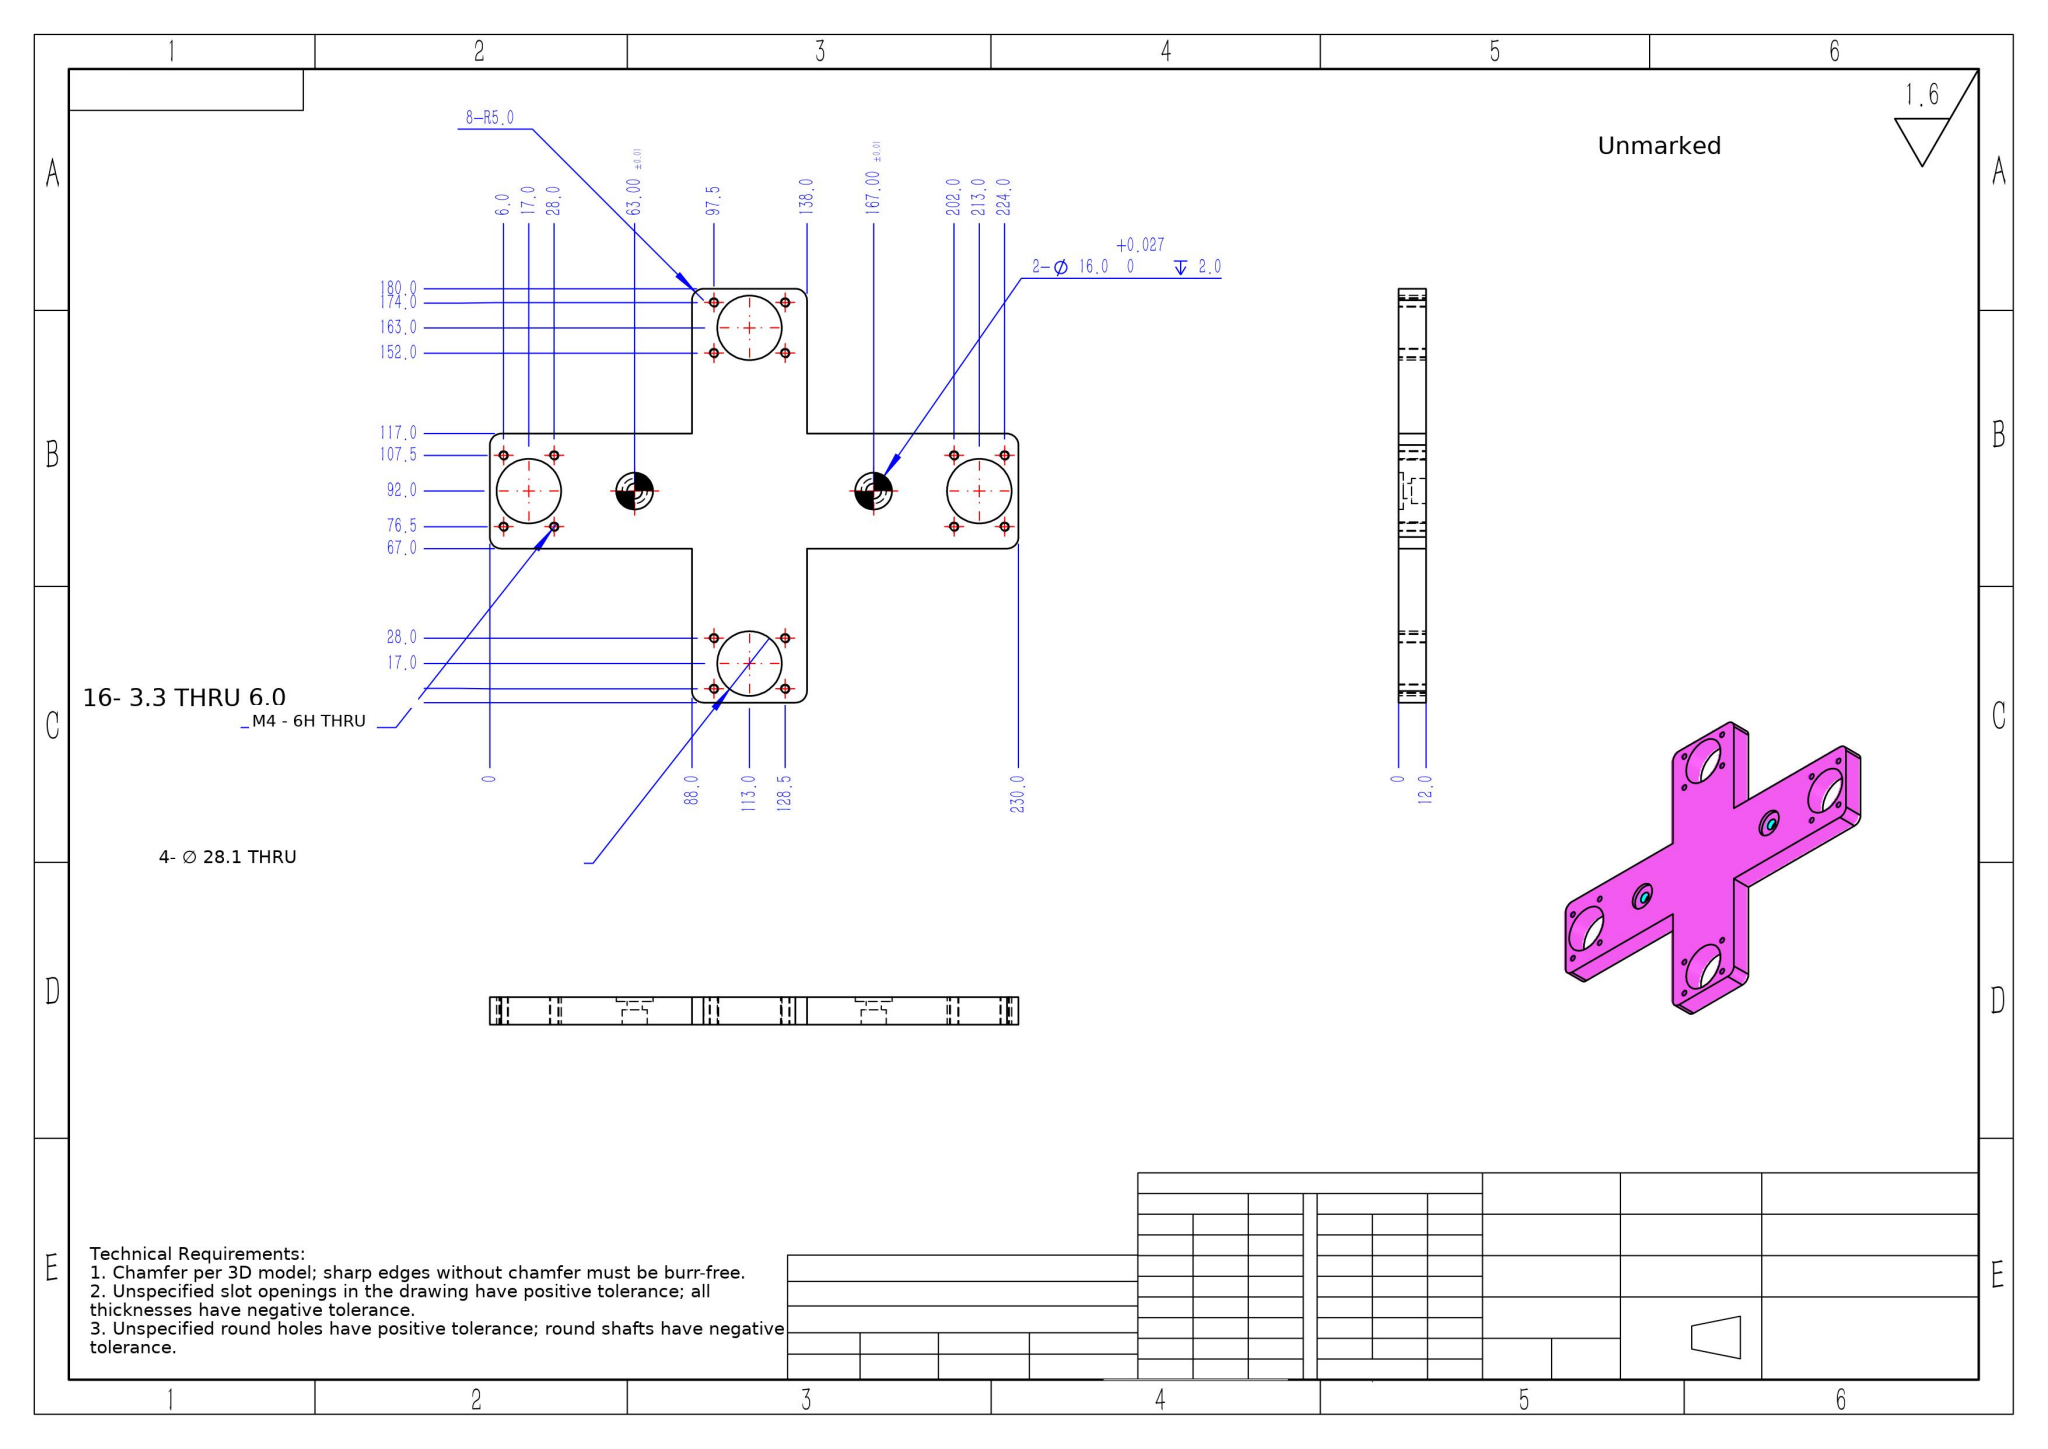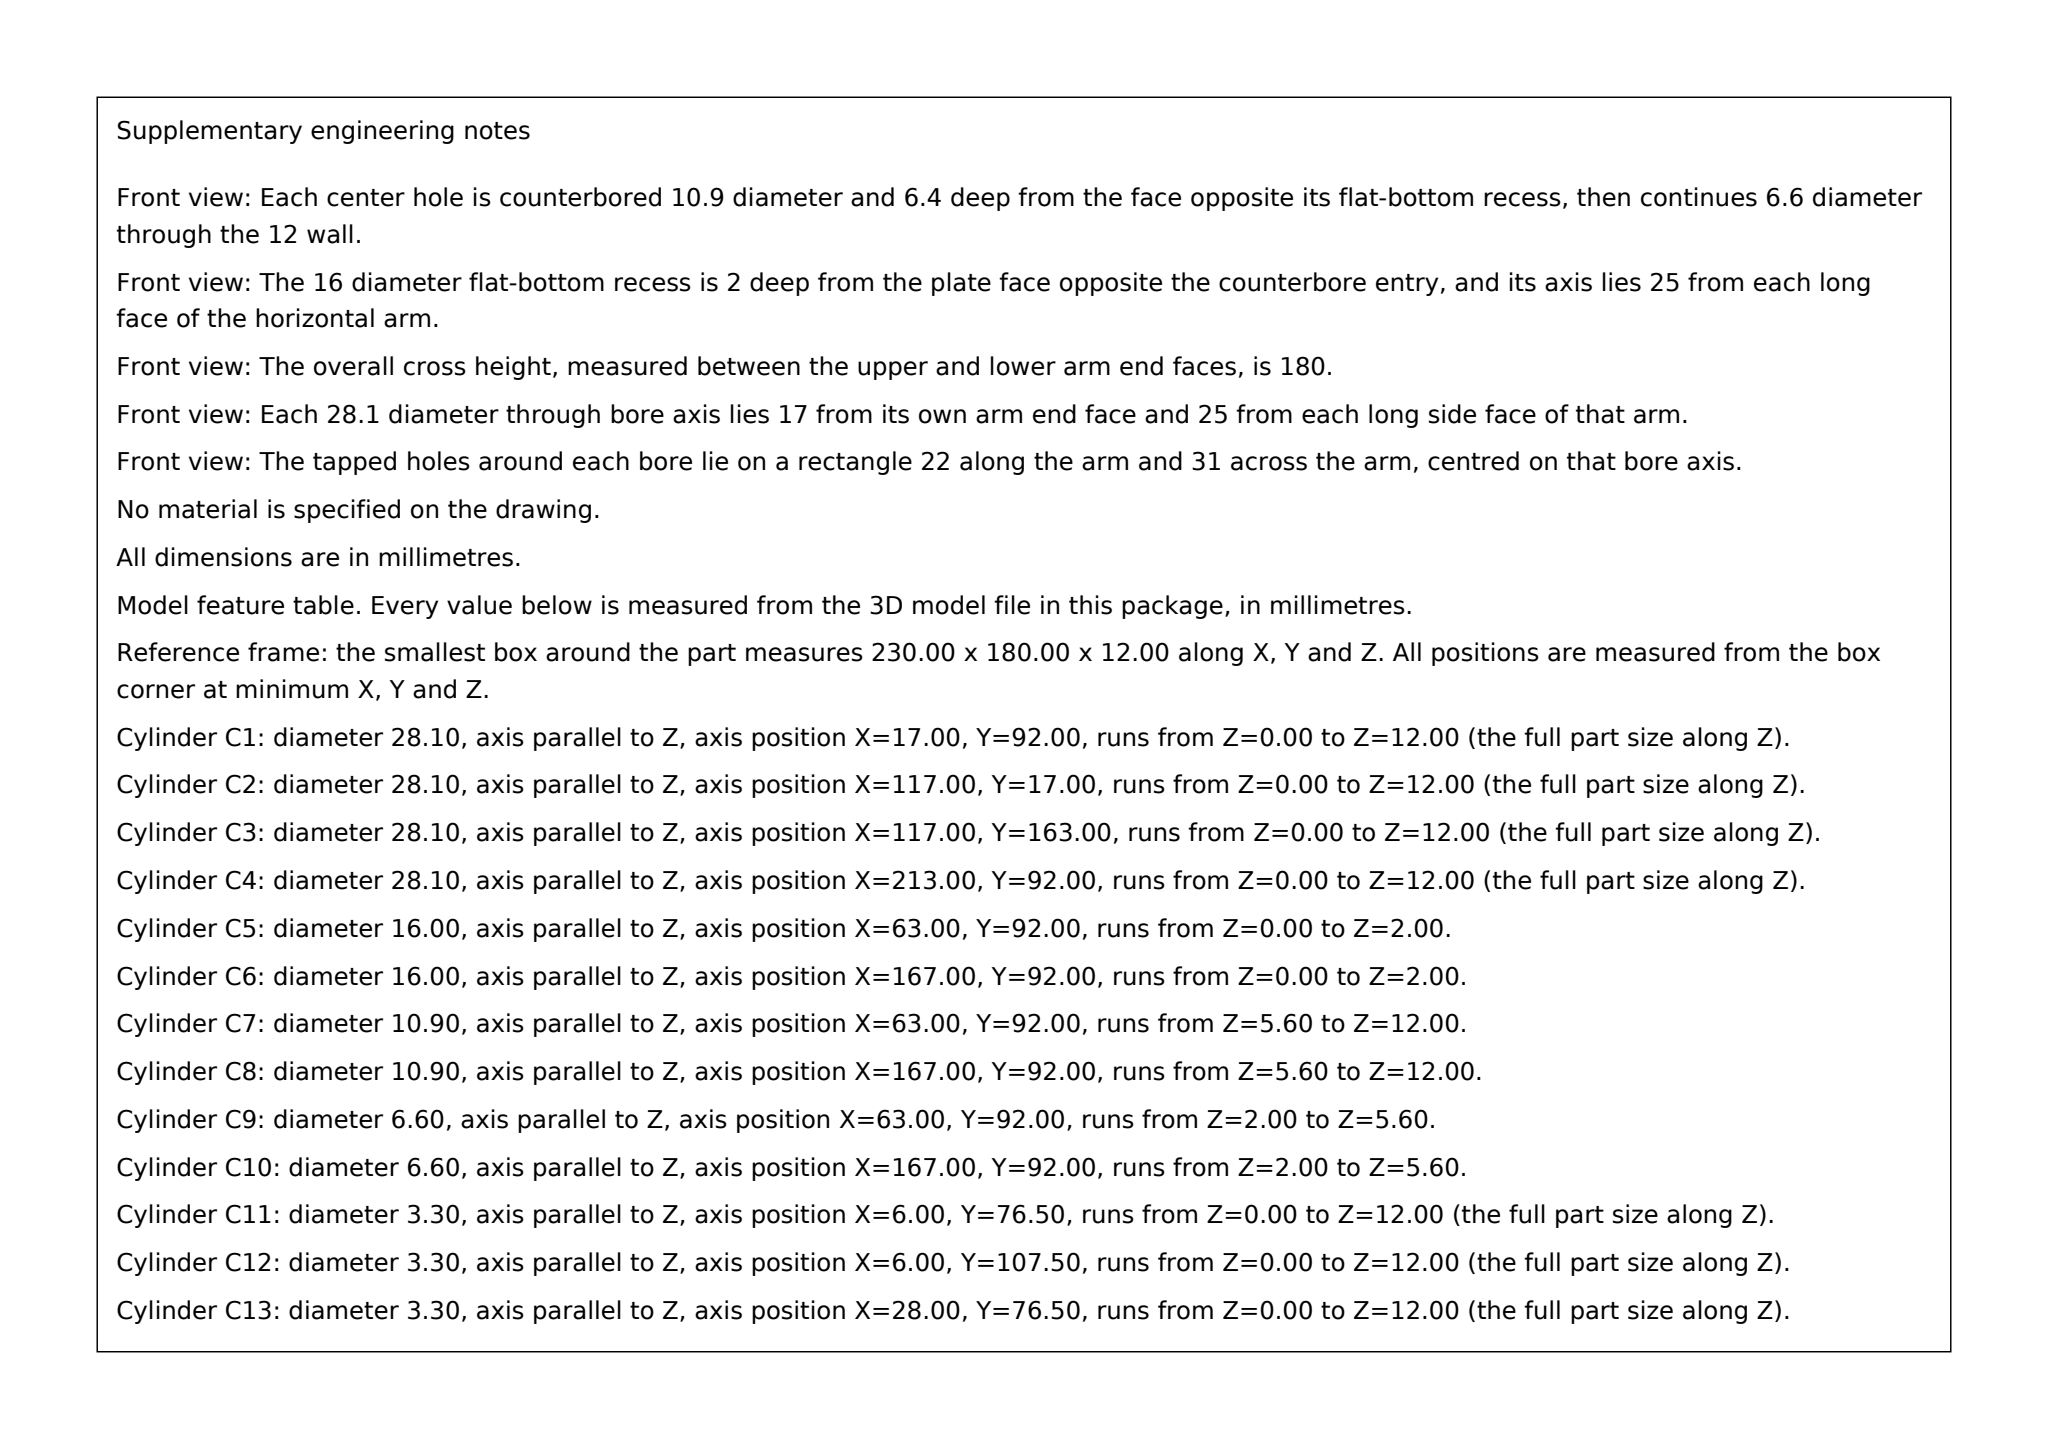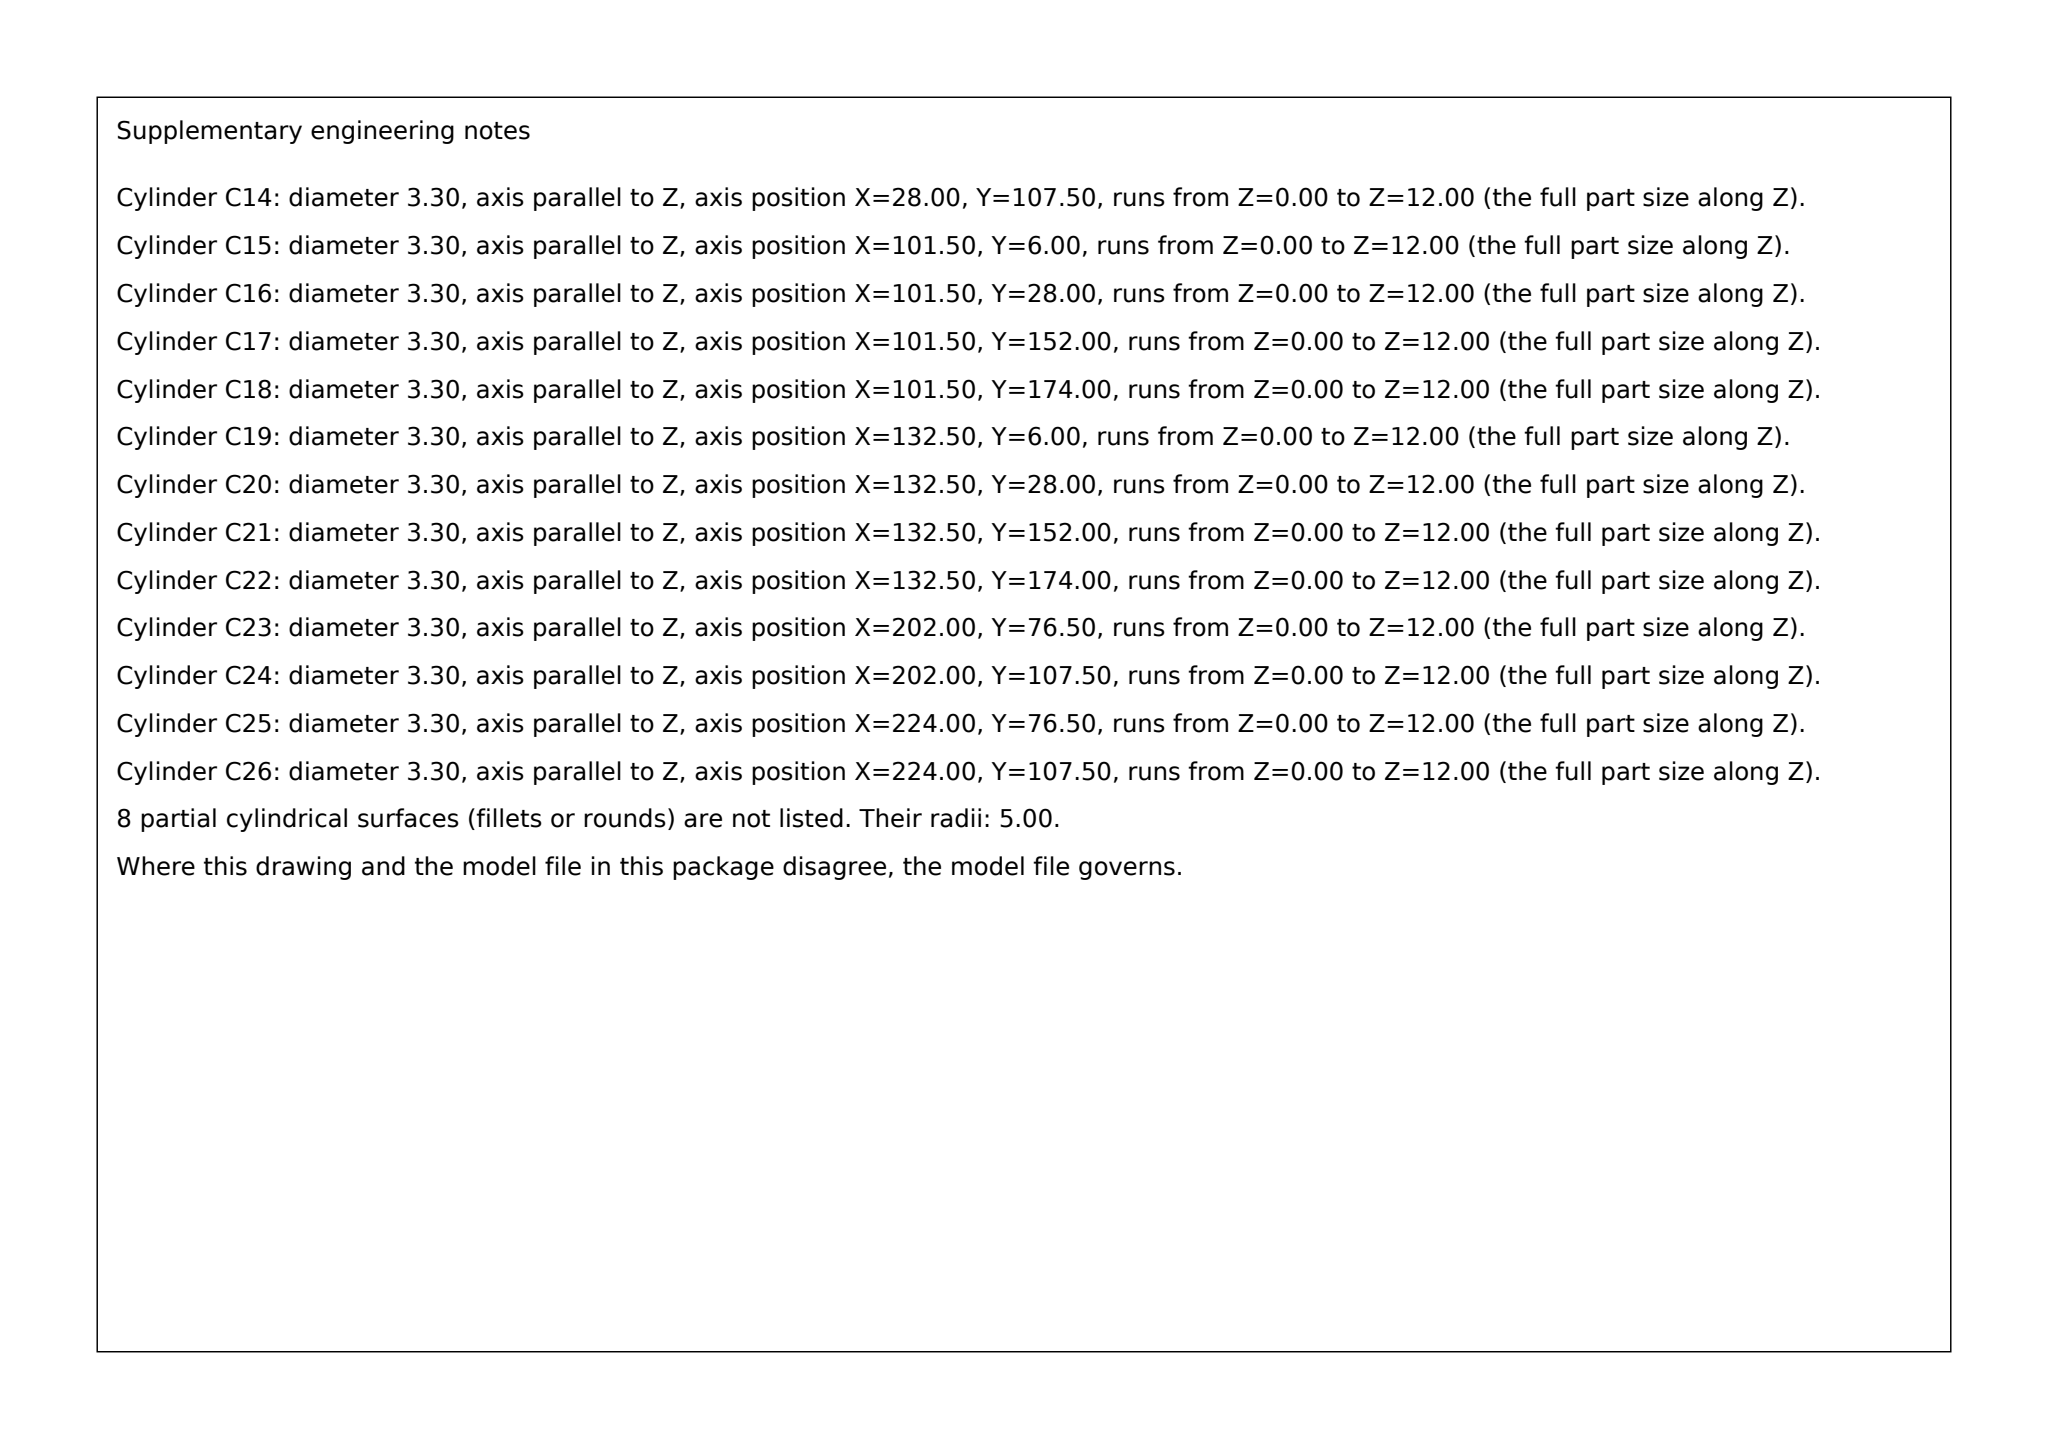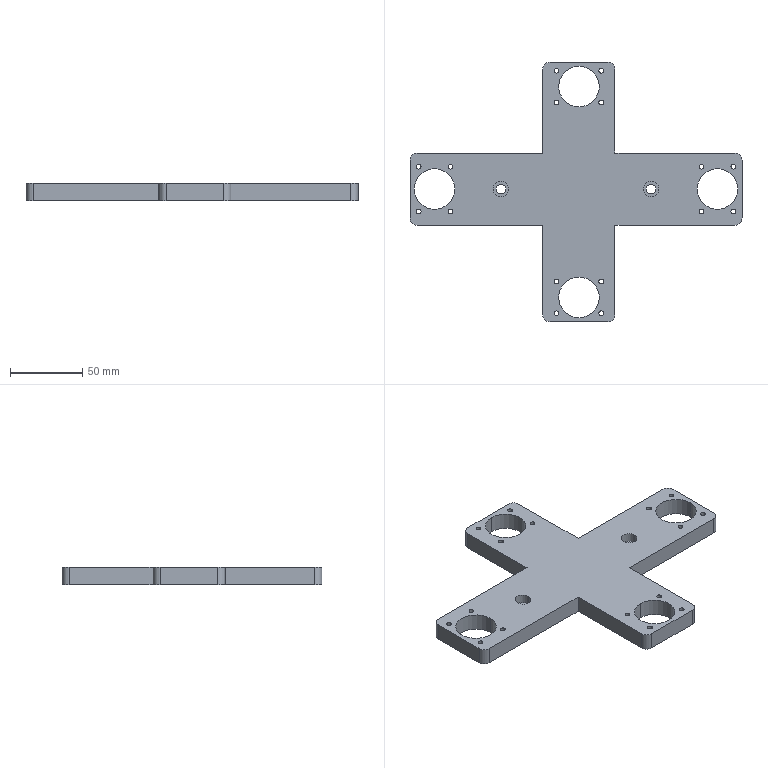Part | SolidWorks | mm | 1 solid | 78 faces | box 230 x 180 x 12 mm | volume 181830 mm3 | cylinder 60 | plane 18 | commonest cylinder face diameters 3.3 x32 28.1 x8 10 x8 10.9 x4 6.6 x4 16 x4
Drawing notes:
VERT ARM 50 WIDE: SIDE FACES X=92 & X=142 FROM LH EDGE | from the solid: axis_planes x=92.0 and x=142.0 within bbox X 0-230 give 50 wide centre arm
4X Ø28.1 THRU AT (17,92)(117,17)(117,163)(213,92) FROM LH/BTM EDGES | from the solid: 28.1 dia z-cylinders at those XY, len 12 = full 12 thk
2X Ø10.9 DP 6.4 FAR SIDE AT (63,92)(167,92) FROM LH/BTM EDGES | from the solid: 10.9 dia z-cylinders at (63,92) and (167,92), depth 6.4 from z=12 face
8X M4-6H IN VERT ARMS AT X=101.5 & 132.5 FROM LEFT EDGE (0) | from the solid: Ø3.3 thru cyls at x=101.5 and x=132.5, y=6.0/28.0/152.0/174.0
LOWER M4-6H ROW AT Y=6.0 FROM BOTTOM EDGE (0) | from the solid: Ø3.3 cyls at (101.5,6.0) and (132.5,6.0); bbox Y=0 at bottom edge